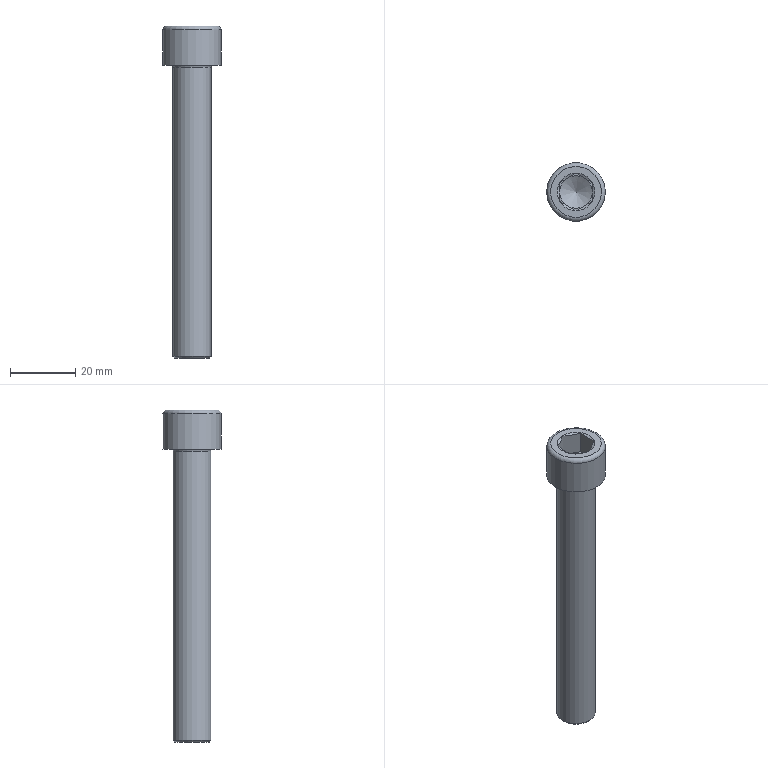Component | NX | SET_SCREW | 1 solid | 27 faces | volume 12009 mm3 | plane 15 | cone 8 | cylinder 2 | torus 2 | commonest cylinder face diameters 11.701 x1 18 x1